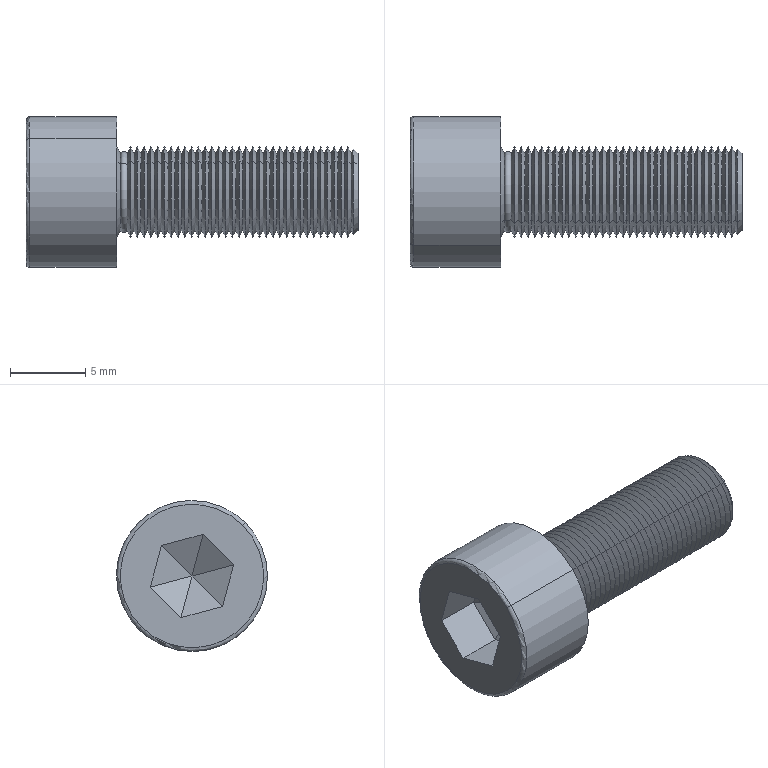Component | SolidWorks | Z24X50X20LockingAssembly-1_000102Z000060016-2 | 1 solid | 172 faces | volume 781 mm3 | cone 148 | plane 16 | torus 4 | cylinder 4 | commonest cylinder face diameters 10 x2 6.012 x2